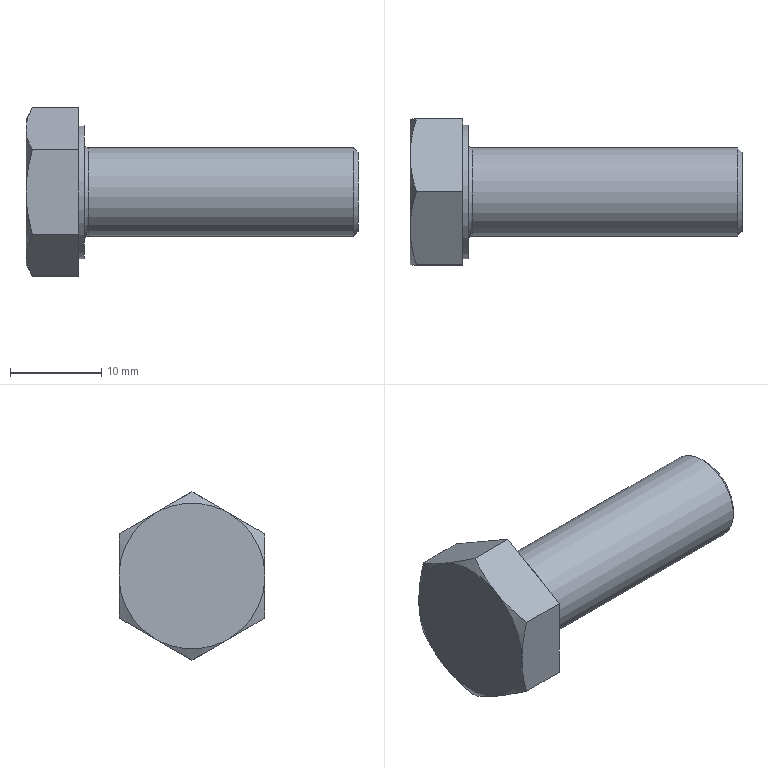Component | NX | GB-T5783-2000_M10X30 | 1 solid | 20 faces | volume 3611 mm3 | plane 10 | cone 7 | cylinder 2 | torus 1 | commonest cylinder face diameters 14.63 x1 9.732 x1